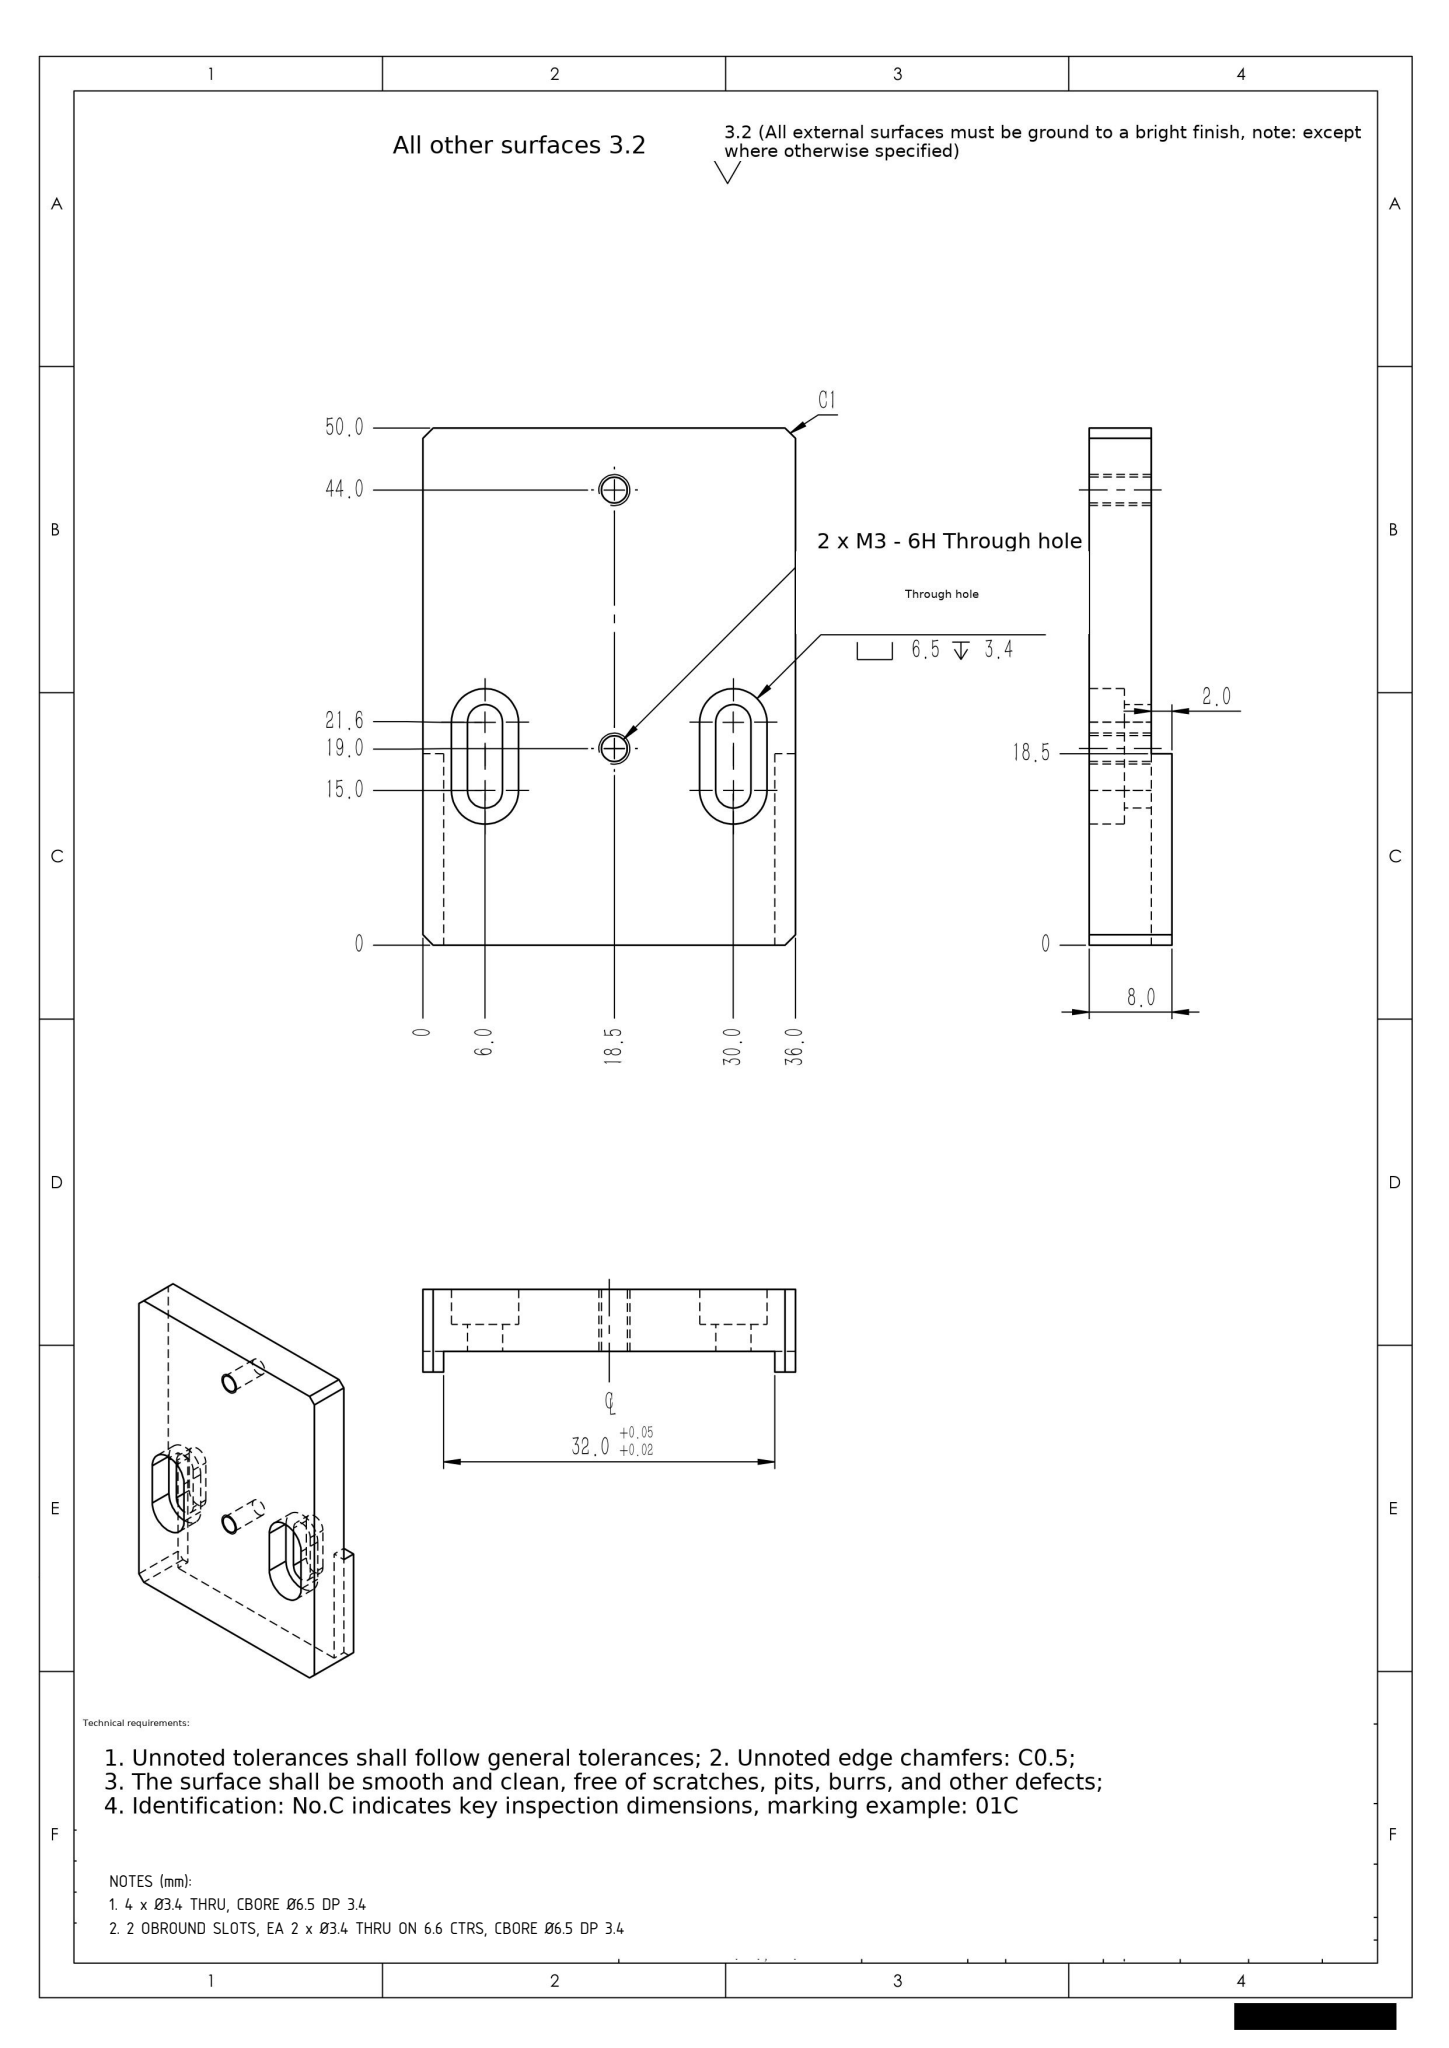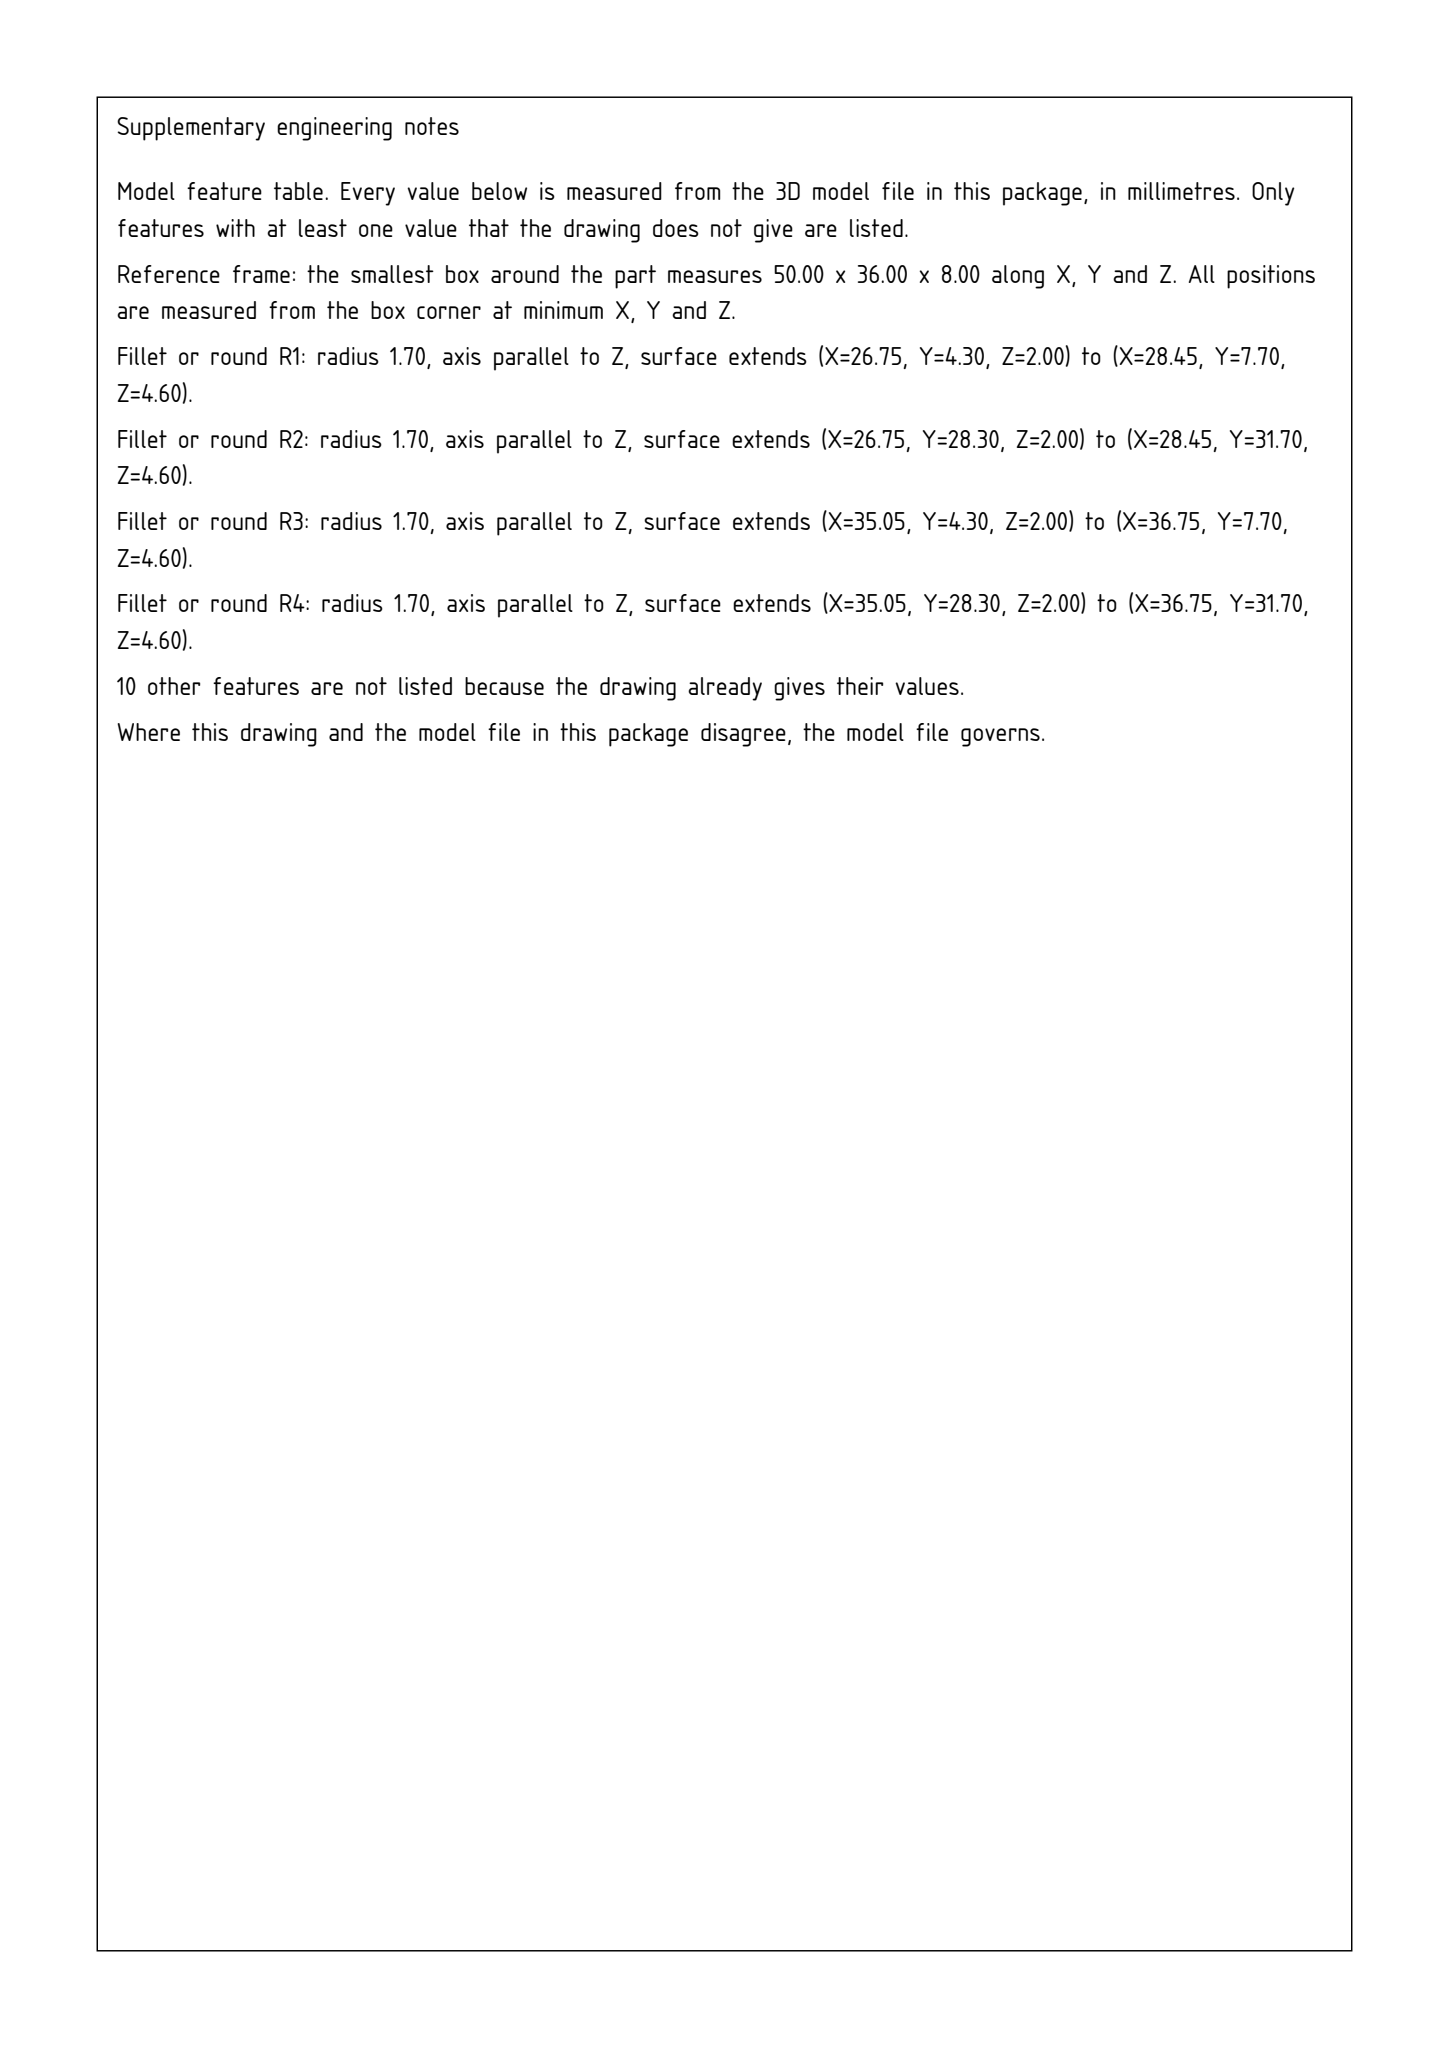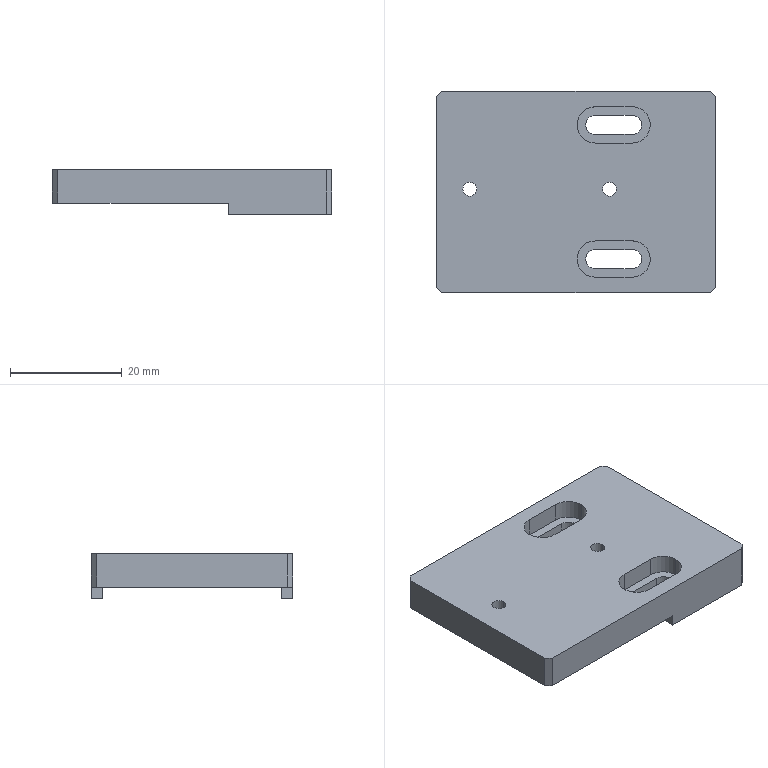Part | SolidWorks | mm | 1 solid | 42 faces | box 50 x 36 x 8 mm | volume 10194 mm3 | plane 26 | cylinder 16 | commonest cylinder face diameters 6.5 x6 3.4 x6 2.5 x4
Drawing notes:
4 x Ø3.4 THRU, CBORE Ø6.5 DP 3.4 | from the solid: Four Ø3.4 cyls len 2.6 at (28.45,6.0),(35.05,6.0),(28.45,30.0),(35.05,30.0) each with coaxial Ø6.5 c'bore depth 3.4
2 OBROUND SLOTS, EA 2 x Ø3.4 THRU ON 6.6 CTRS, CBORE Ø6.5 DP 3.4 | from the solid: Pairs of Ø3.4 holes at x=28.45 & 35.05 (6.6 apart) on y=6.0 and y=30.0; Ø6.5 c'bores depth 3.4